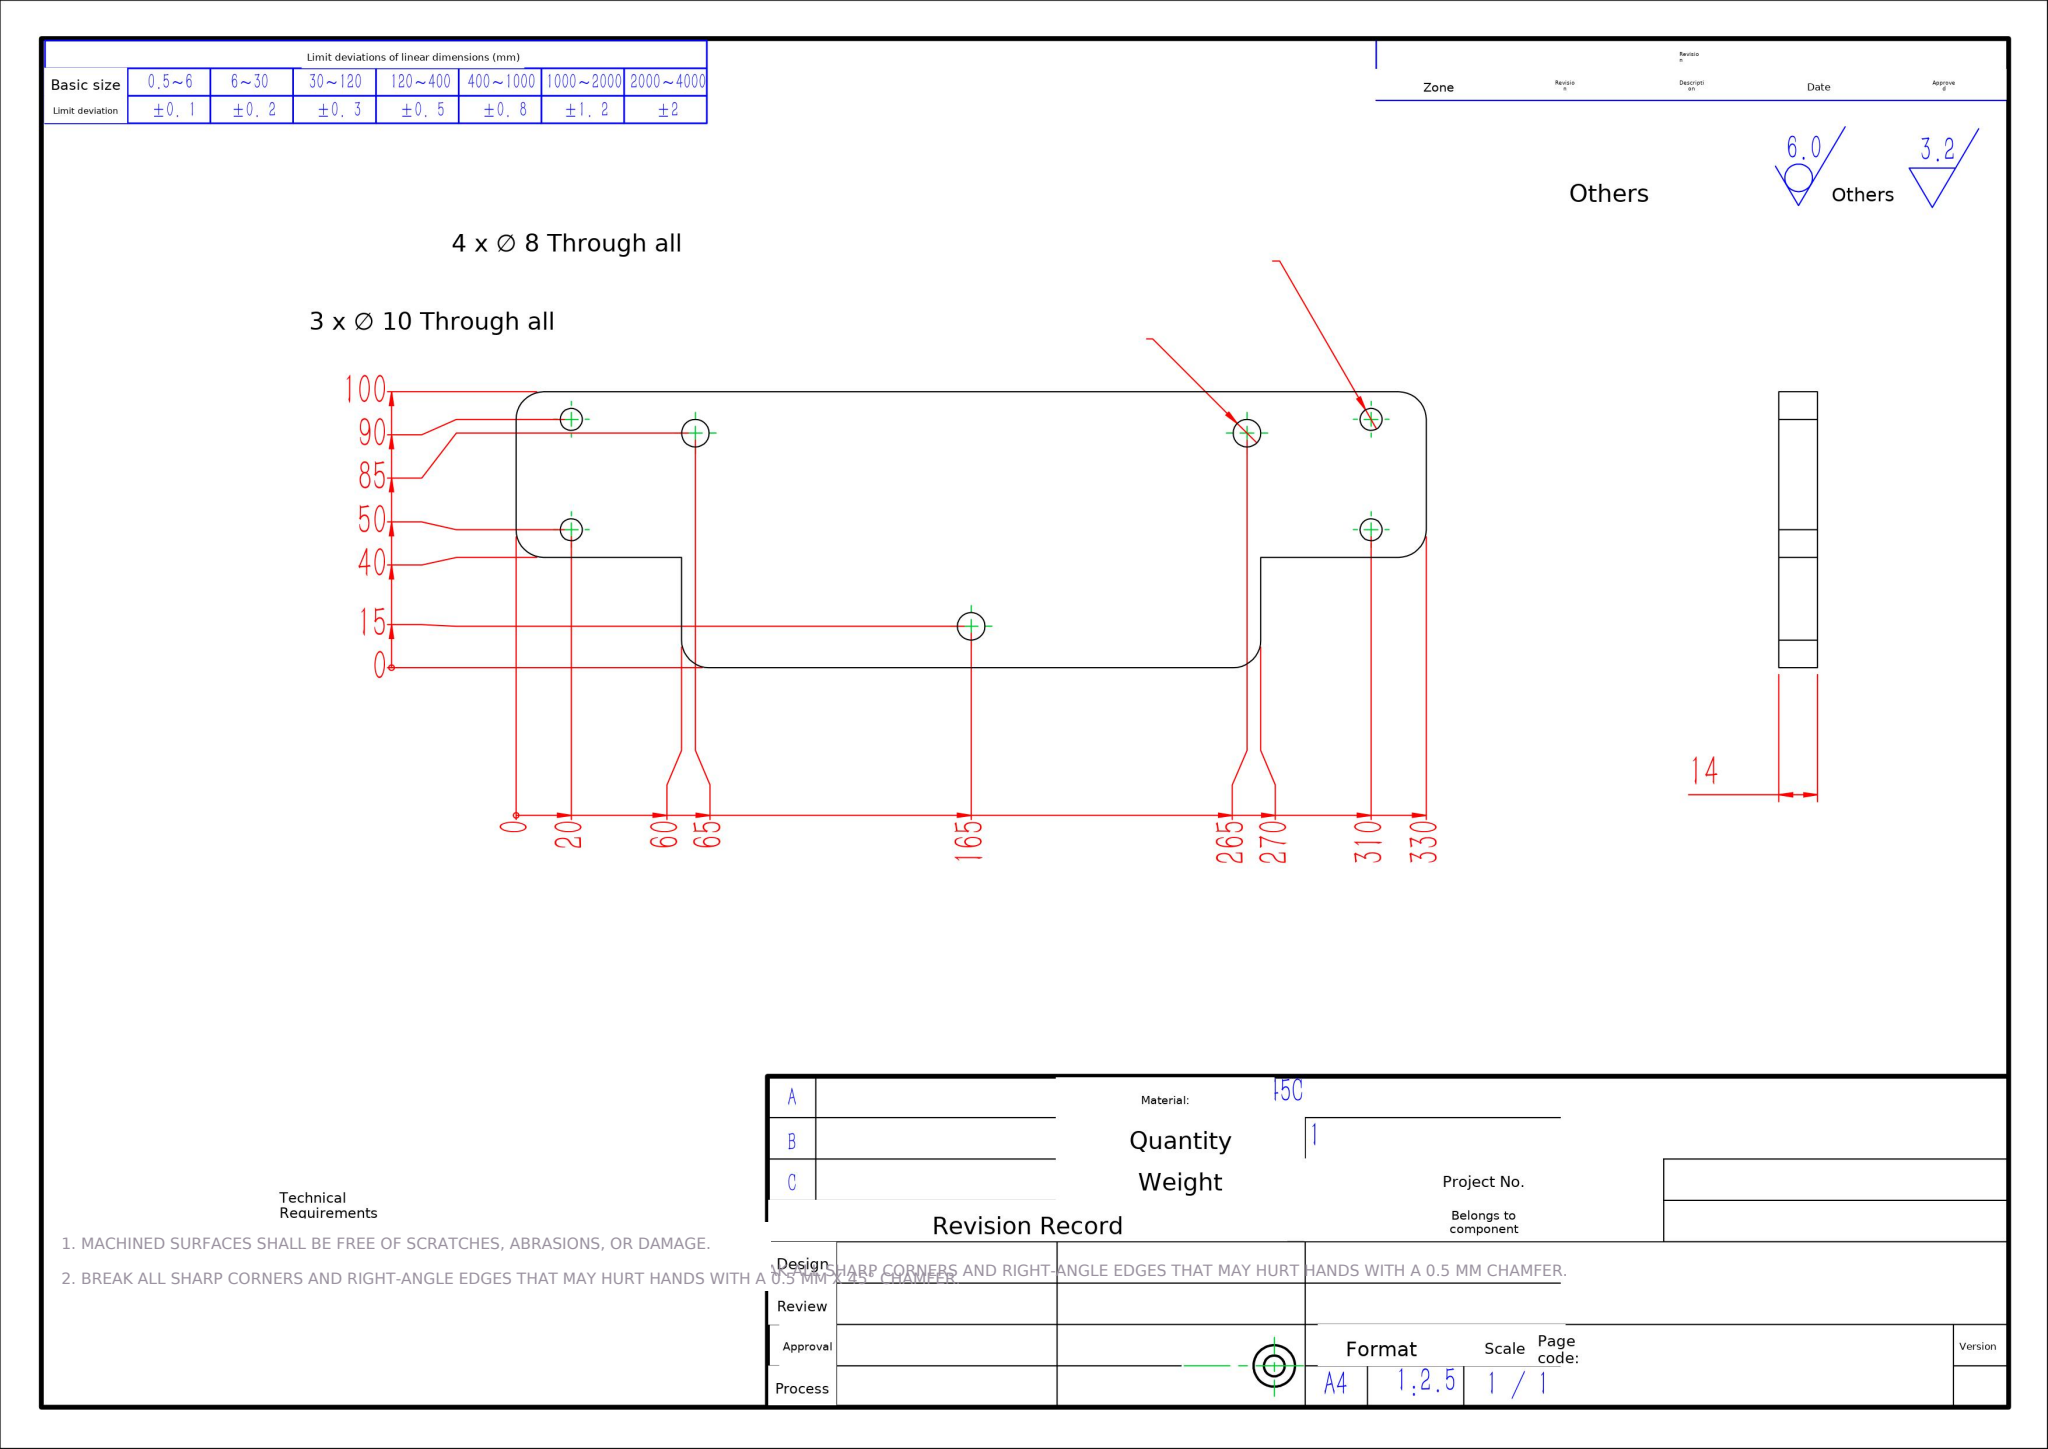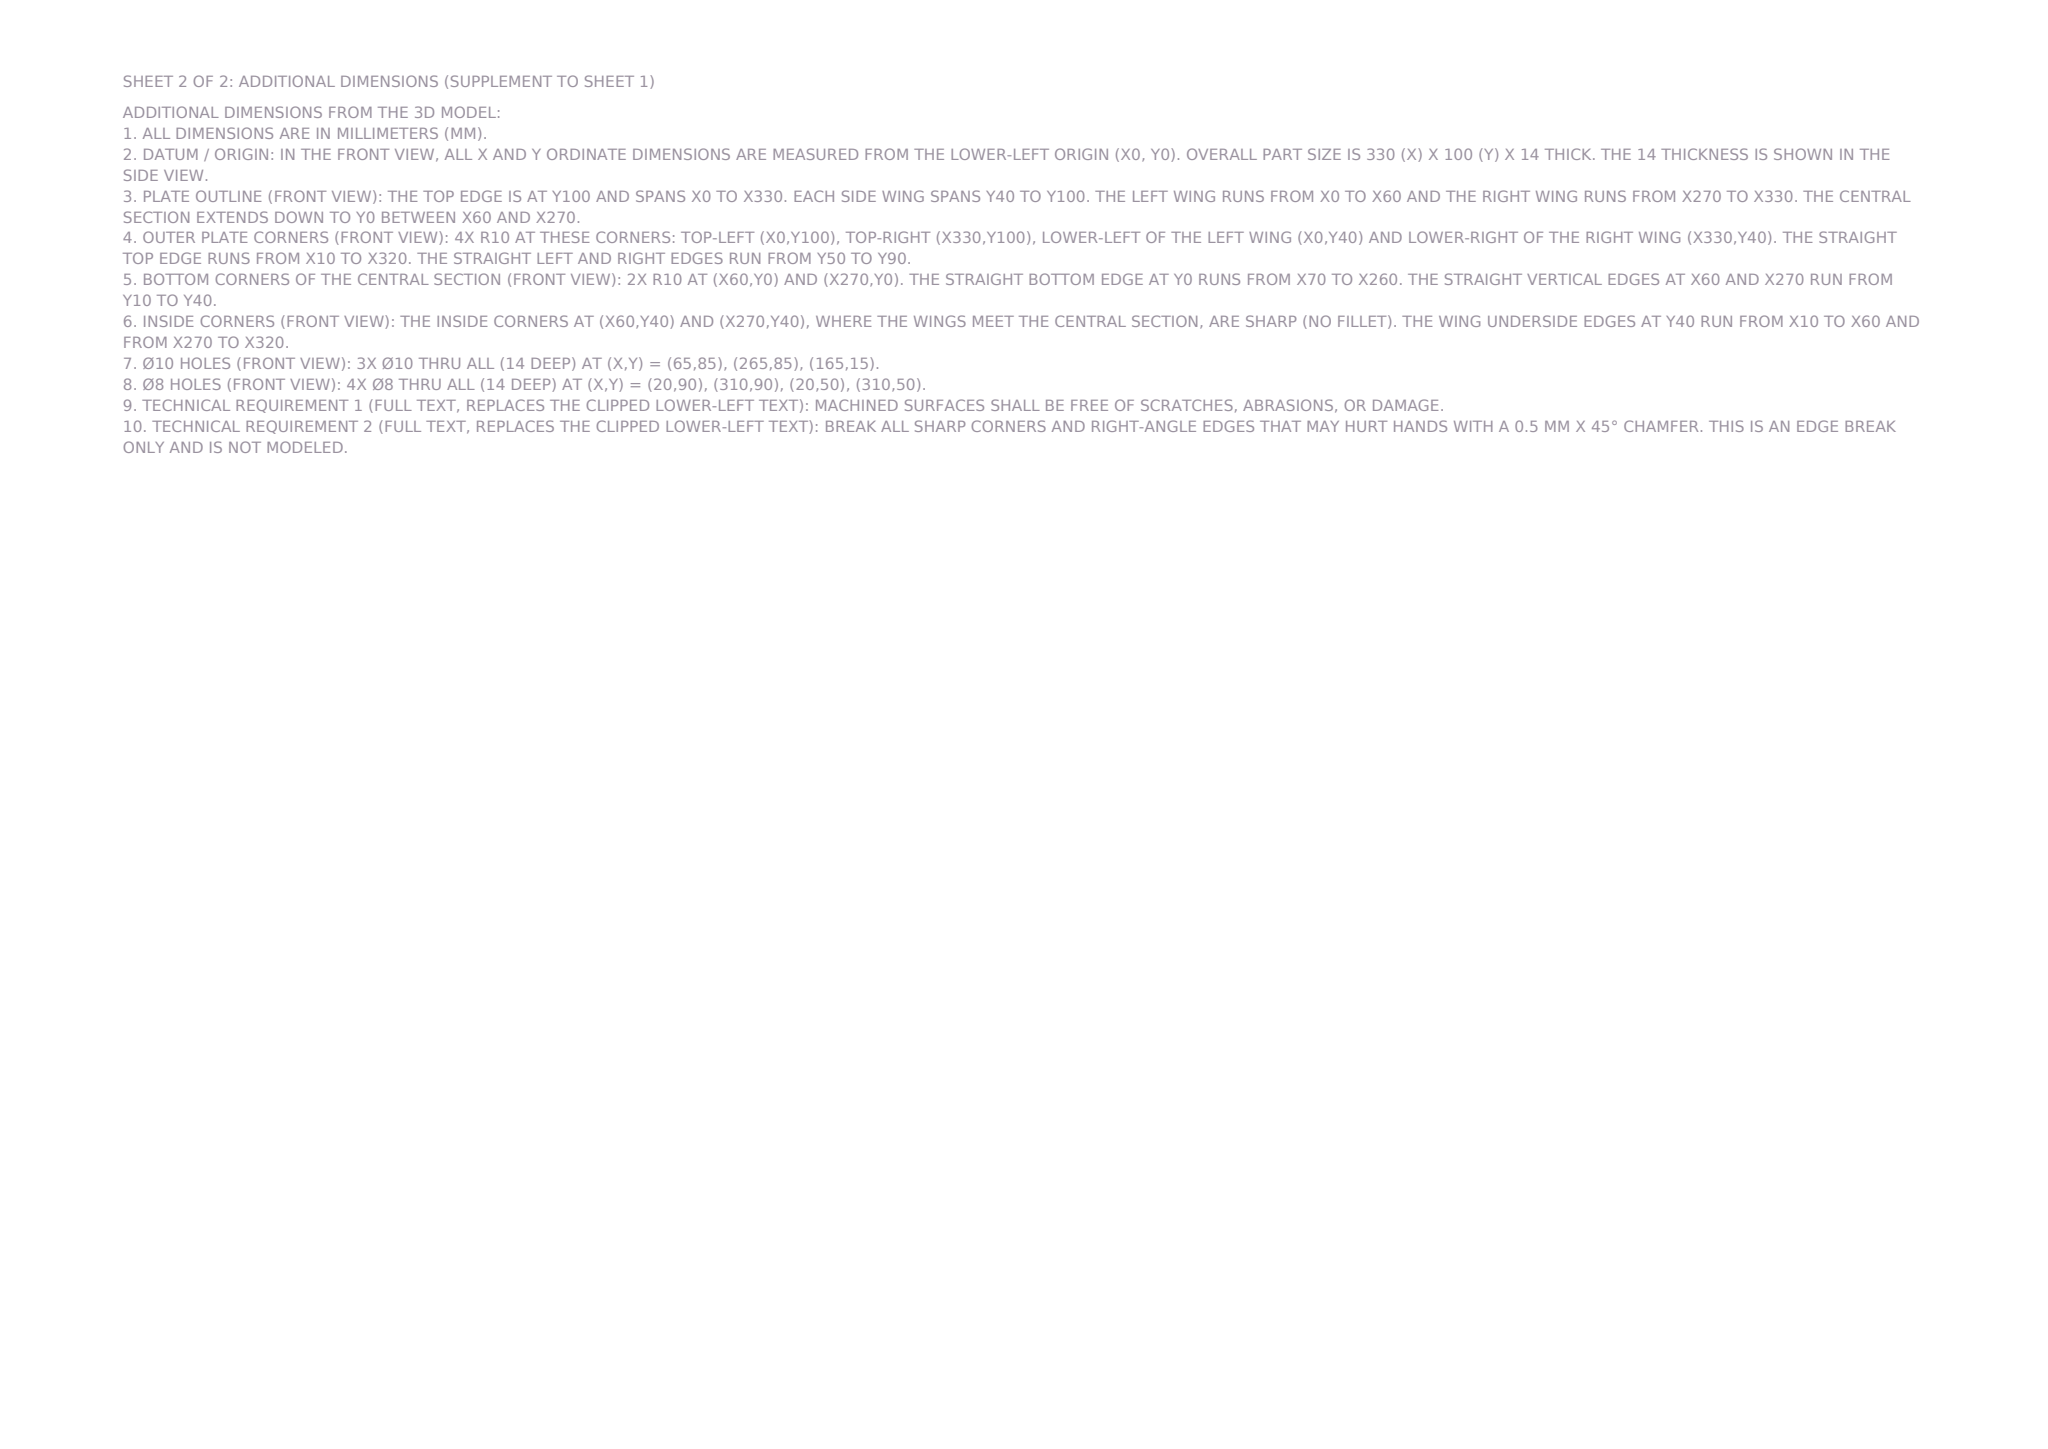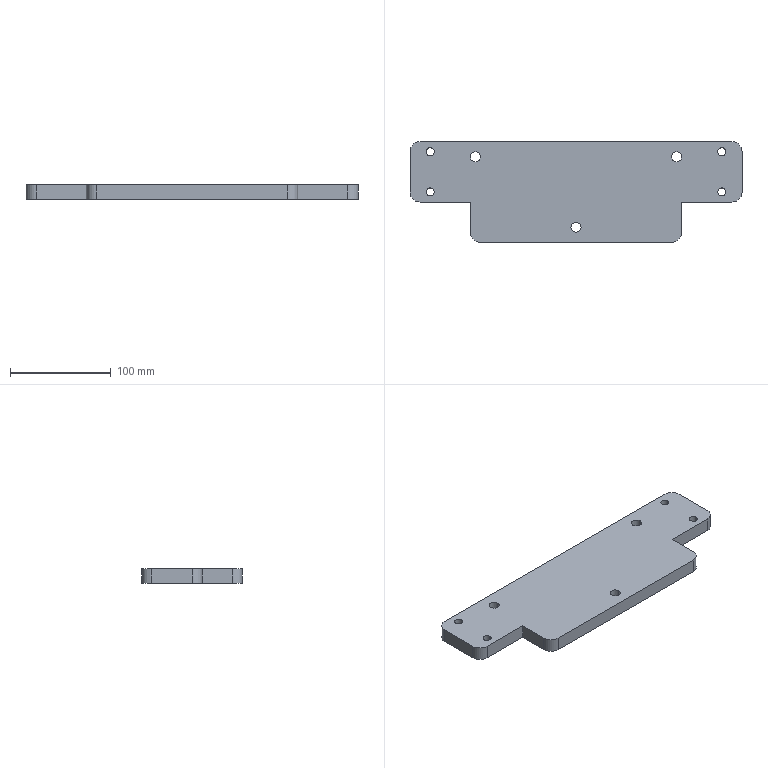Part | NX | mm | 1 solid | 30 faces | box 330 x 100 x 14 mm | volume 386884 mm3 | cylinder 20 | plane 10 | commonest cylinder face diameters 8 x8 10 x6 20 x6